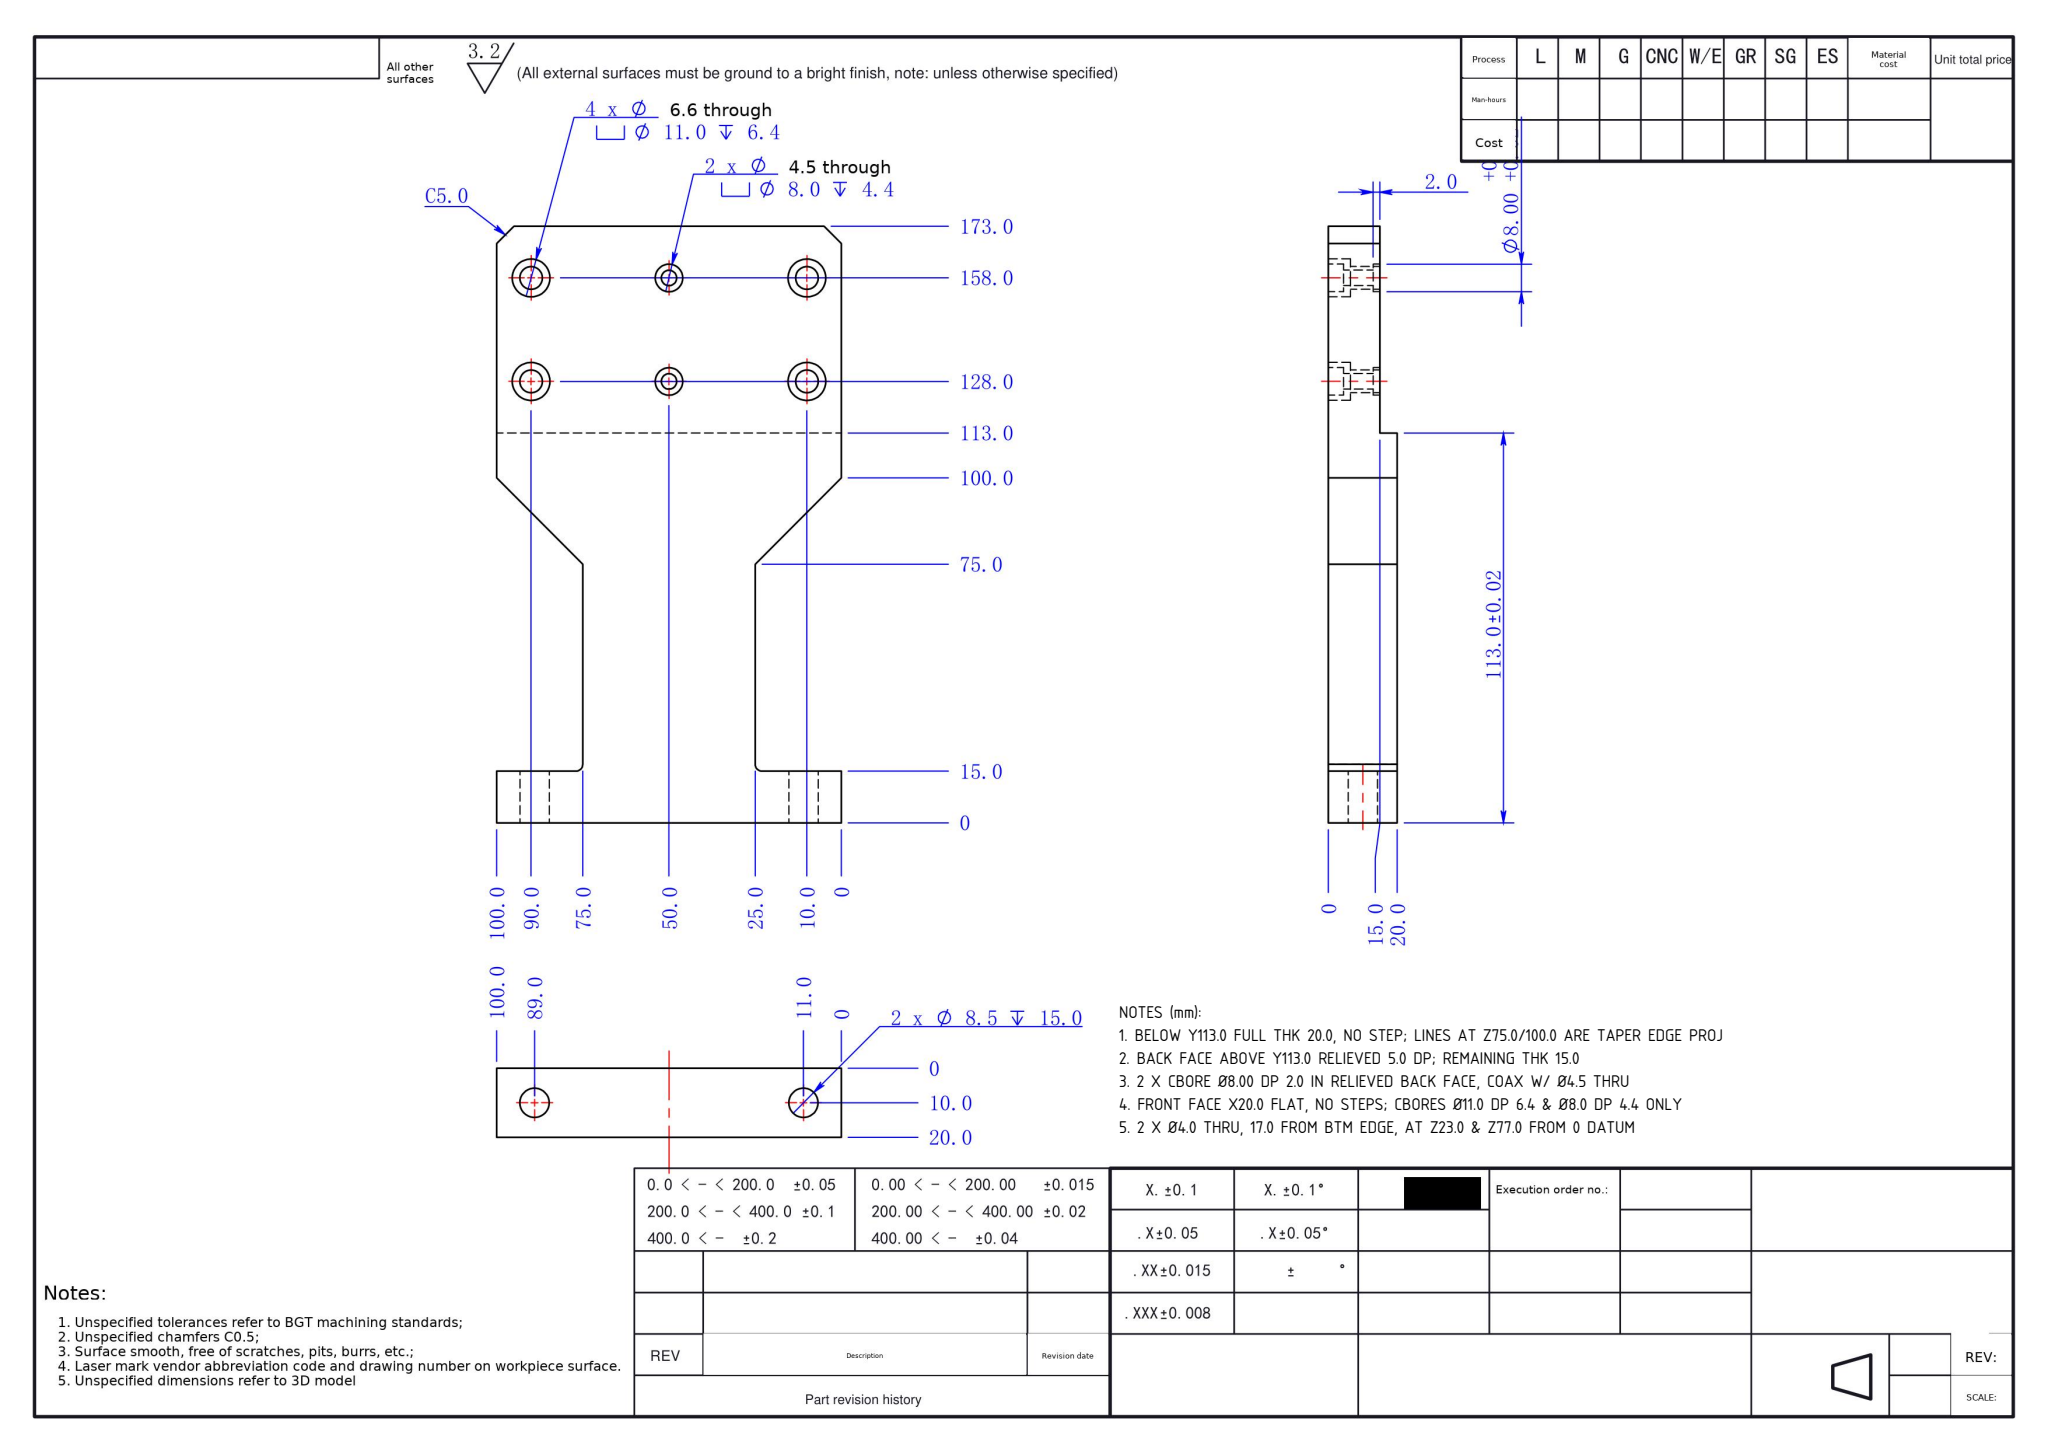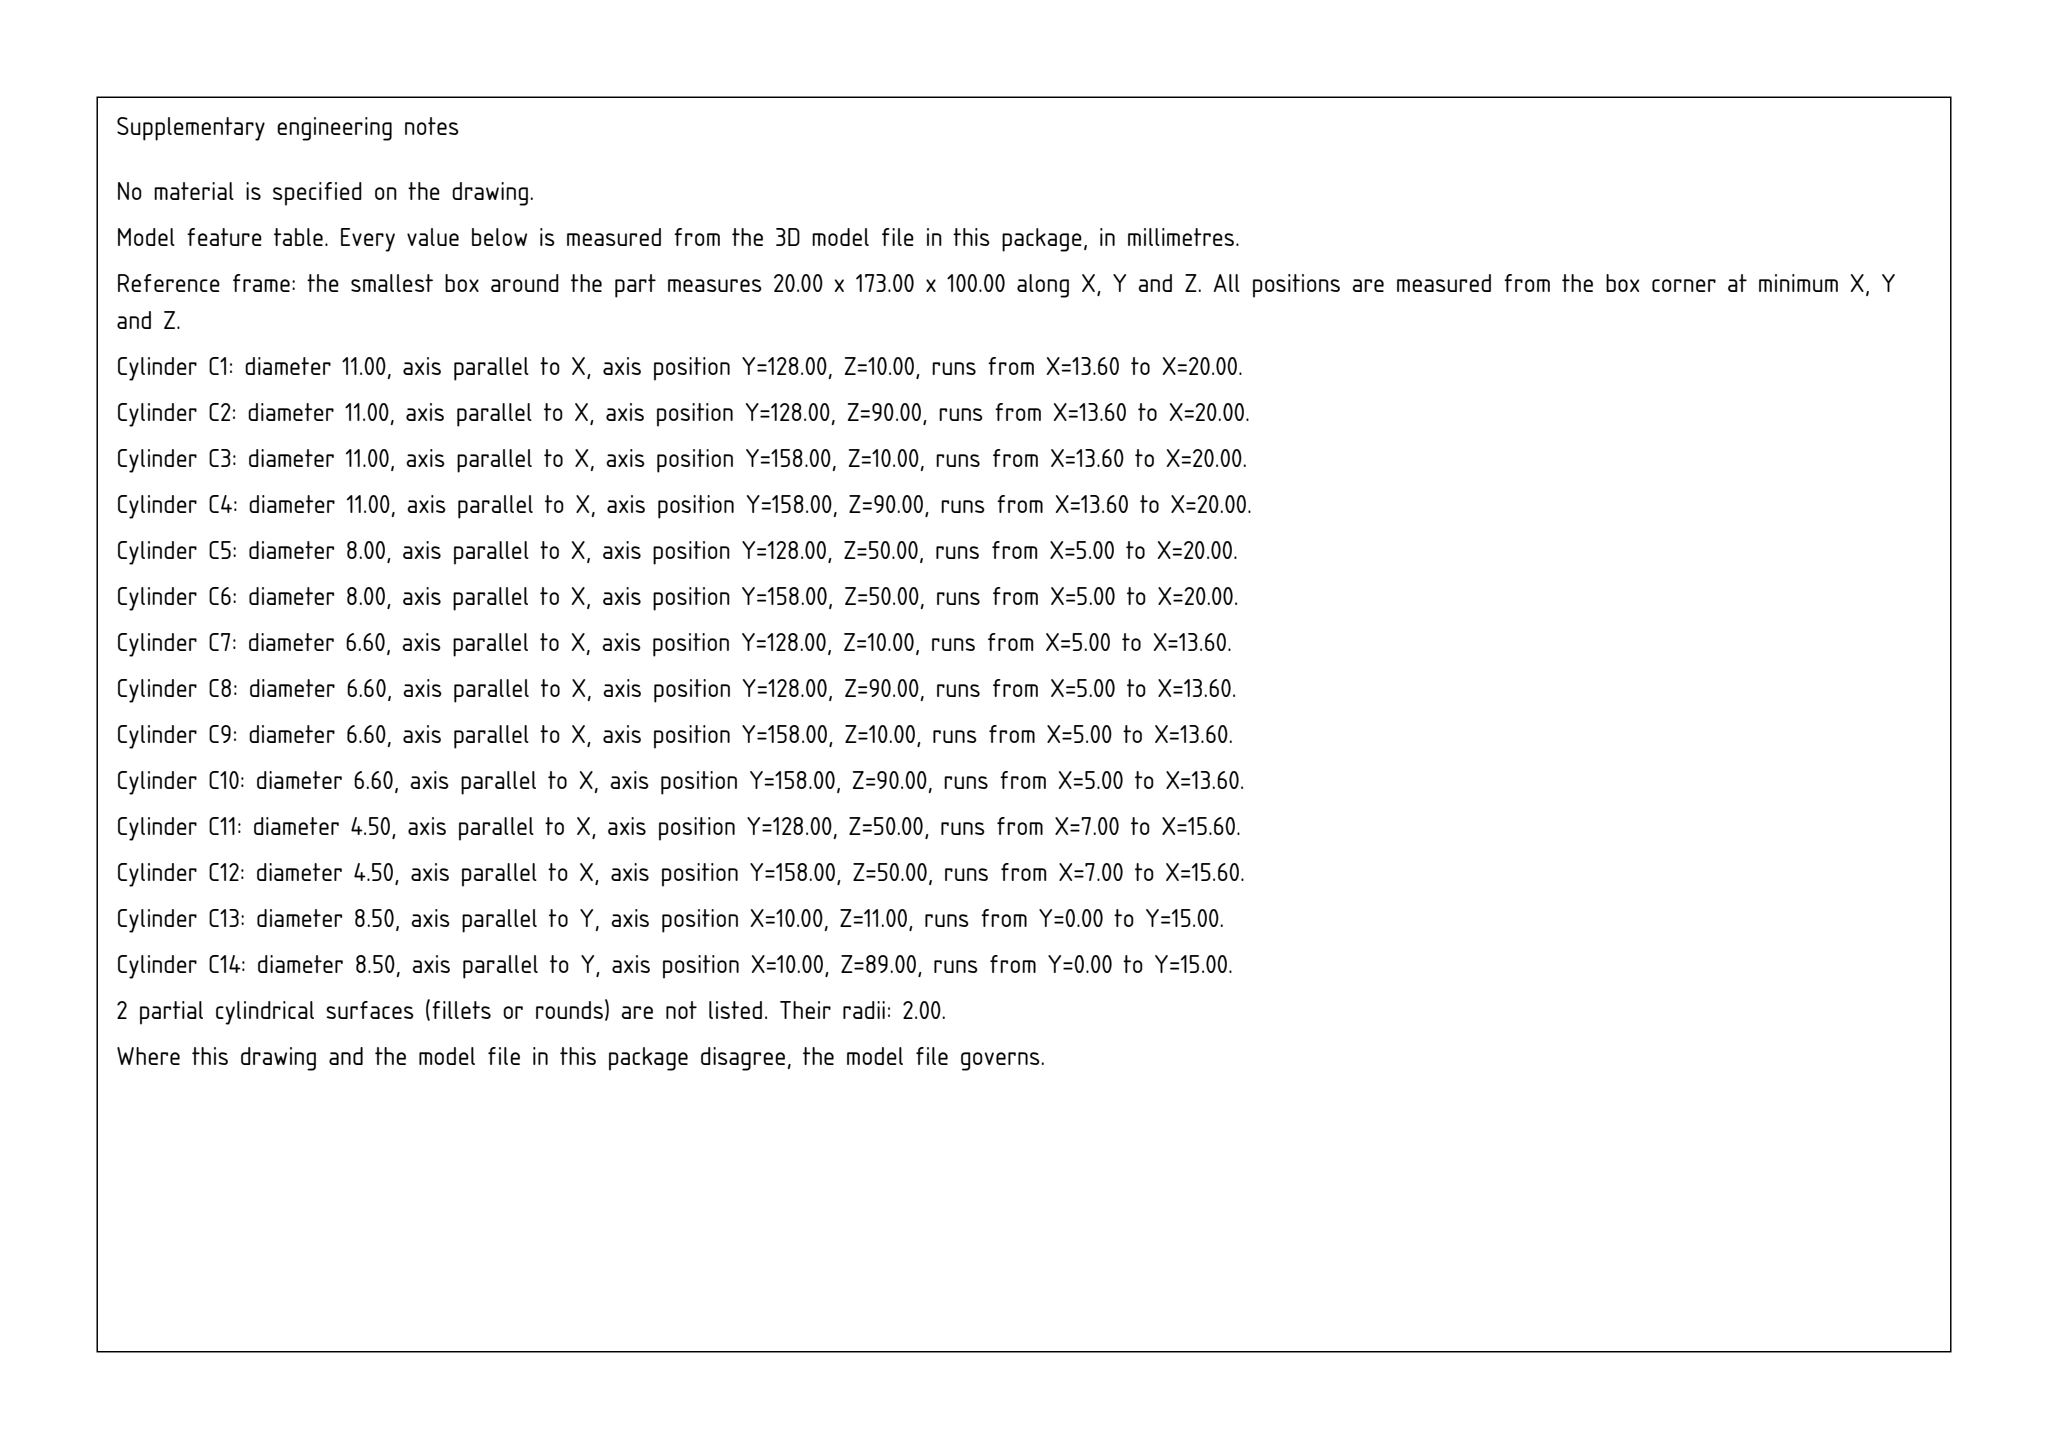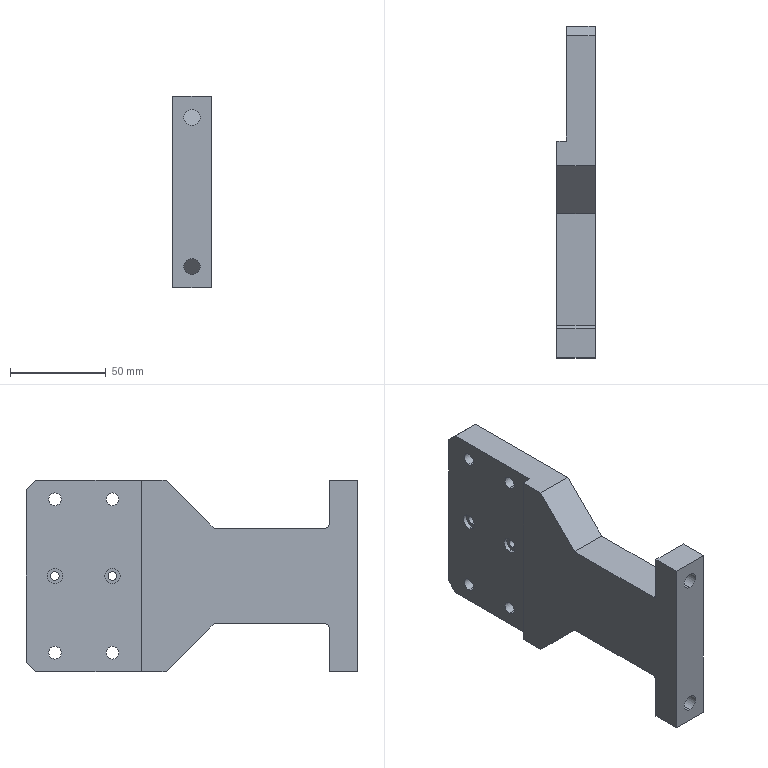Part | SolidWorks | mm | 1 solid | 60 faces | box 20 x 173 x 100 mm | volume 236930 mm3 | cylinder 34 | plane 26 | commonest cylinder face diameters 8 x8 11 x8 6.6 x8 8.5 x4 4.5 x4 4 x2
Drawing notes:
BELOW Y113.0 FULL THK 20.0, NO STEP; LINES AT Z75.0/100.0 ARE TAPER EDGE PROJ | from the solid: z-planes 0,25,75,100 with y-planes 15,113 define tapered profile; no x-plane change below y=113
BACK FACE ABOVE Y113.0 RELIEVED 5.0 DP; REMAINING THK 15.0 | from the solid: x-planes at 0 (y<113 face) and 5.0 (face above y=113); 20-5=15 thk; 6.6 thru L8.6 + cbore 6.4 = 15.0
2 X CBORE Ø8.00 DP 2.0 IN RELIEVED BACK FACE, COAX W/ Ø4.5 THRU | from the solid: cyl Ø8.0 L2.0 at (y=128,z=50) & (y=158,z=50), x 5.0 to 7.0 (x-plane 7.0 count 2)
FRONT FACE X20.0 FLAT, NO STEPS; CBORES Ø11.0 DP 6.4 & Ø8.0 DP 4.4 ONLY | from the solid: only x-planes 13.6 (=20-6.4, 4 off) and 15.6 (=20-4.4, 2 off) behind x=20 face
2 X Ø4.0 THRU, 17.0 FROM BTM EDGE, AT Z23.0 & Z77.0 FROM 0 DATUM | from the solid: cylinders Ø4.0 axis x at (y=17.0,z=23.0) and (y=17.0,z=77.0), length 20.0 = full THK